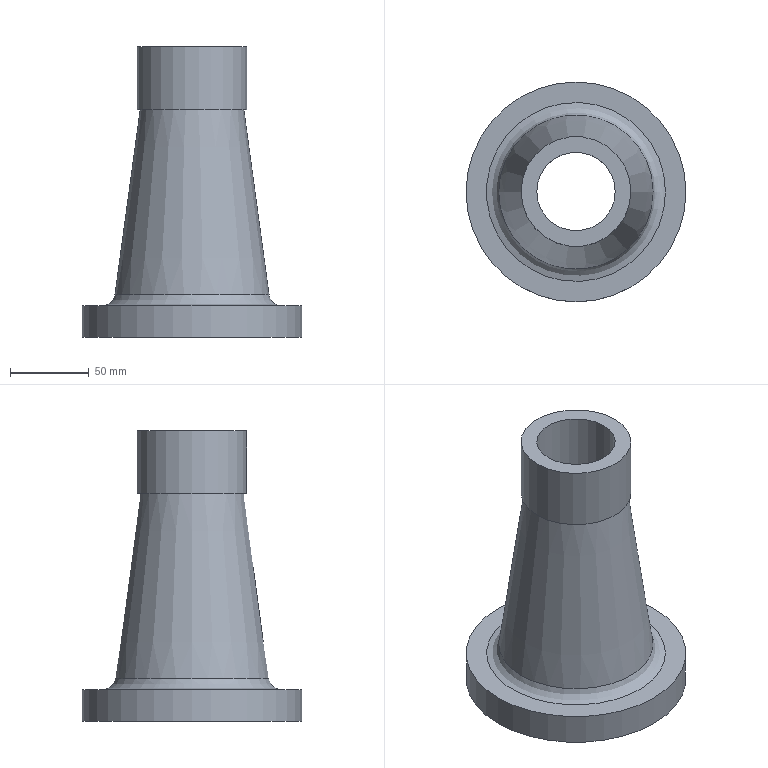Component | NX | BODY | 1 solid | 12 faces | box 140 x 140 x 185 mm | volume 559326 mm3 | plane 5 | cylinder 4 | cone 2 | torus 1 | commonest cylinder face diameters 100 x1 140 x1 70 x1 50 x1
STEP:
#1=CARTESIAN_POINT('',(0.,0.,0.));
#2=DIRECTION('',(0.,0.,1.));
#3=DIRECTION('',(1.,0.,0.));
#4=AXIS2_PLACEMENT_3D('',#1,#2,#3);
#5=CARTESIAN_POINT('',(-42.22,240.,3.));
#6=VERTEX_POINT('',#5);
#7=CARTESIAN_POINT('',(0.,240.,3.));
#8=DIRECTION('',(0.,0.,-1.));
#9=DIRECTION('',(-1.,0.,0.));
#10=AXIS2_PLACEMENT_3D('',#7,#8,#9);
#11=CIRCLE('',#10,42.22);
#12=CARTESIAN_POINT('',(0.,240.,129.617));
#13=DIRECTION('',(0.,0.,-1.));
#14=DIRECTION('',(-1.,0.,0.));
#15=AXIS2_PLACEMENT_3D('',#12,#13,#14);
#16=CONICAL_SURFACE('',#15,25.,0.1352);
#17=CARTESIAN_POINT('',(0.,126.617));
#18=DIRECTION('',(1.,0.));
#19=VECTOR('',#18,1.);
#20=LINE('',#17,#19);
#21=(GEOMETRIC_REPRESENTATION_CONTEXT(2)PARAMETRIC_REPRESENTATION_CONTEXT()REPRESENTATION_CONTEXT('',''));
#22=DEFINITIONAL_REPRESENTATION('',(#20),#21);
#23=PCURVE('',#16,#22);
#24=CARTESIAN_POINT('',(0.,282.22,3.));
#25=DIRECTION('',(0.,0.,-1.));
#26=DIRECTION('',(-1.,0.,0.));
#27=AXIS2_PLACEMENT_3D('',#24,#25,#26);
#28=PLANE('',#27);
#29=CARTESIAN_POINT('',(0.,-42.22));
#30=DIRECTION('',(1.,0.));
#31=AXIS2_PLACEMENT_2D('',#29,#30);
#32=CIRCLE('',#31,42.22);
#33=(GEOMETRIC_REPRESENTATION_CONTEXT(2)PARAMETRIC_REPRESENTATION_CONTEXT()REPRESENTATION_CONTEXT('',''));
#34=DEFINITIONAL_REPRESENTATION('',(#32),#33);
#35=PCURVE('',#28,#34);
#36=SURFACE_CURVE('',#11,(#23,#35),.PCURVE_S1.);
#37=EDGE_CURVE('',#6,#6,#36,.T.);
#38=ORIENTED_EDGE('',*,*,#37,.F.);
#39=CARTESIAN_POINT('',(-25.,240.,129.617));
#40=VERTEX_POINT('',#39);
#41=CARTESIAN_POINT('',(-25.,240.,129.617));
#42=CARTESIAN_POINT('',(-42.22,240.,3.));
#43=B_SPLINE_CURVE_WITH_KNOTS('',1,(#41,#42),.UNSPECIFIED.,.F.,.F.,(2,2),(0.,127.783),.PIECEWISE_BEZIER_KNOTS.);
#44=CARTESIAN_POINT('',(0.,0.));
#45=DIRECTION('',(0.,1.));
#46=VECTOR('',#45,1.);
#47=LINE('',#44,#46);
#48=(GEOMETRIC_REPRESENTATION_CONTEXT(2)PARAMETRIC_REPRESENTATION_CONTEXT()REPRESENTATION_CONTEXT('',''));
#49=DEFINITIONAL_REPRESENTATION('',(#47),#48);
#50=PCURVE('',#16,#49);
#51=CARTESIAN_POINT('',(6.283,0.));
#52=DIRECTION('',(0.,1.));
#53=VECTOR('',#52,1.);
#54=LINE('',#51,#53);
#55=(GEOMETRIC_REPRESENTATION_CONTEXT(2)PARAMETRIC_REPRESENTATION_CONTEXT()REPRESENTATION_CONTEXT('',''));
#56=DEFINITIONAL_REPRESENTATION('',(#54),#55);
#57=PCURVE('',#16,#56);
#58=SEAM_CURVE('',#43,(#50,#57),.PCURVE_S1.);
#59=EDGE_CURVE('',#40,#6,#58,.T.);
#60=ORIENTED_EDGE('',*,*,#59,.F.);
#61=CARTESIAN_POINT('',(0.,240.,129.617));
#62=DIRECTION('',(0.,0.,-1.));
#63=DIRECTION('',(-1.,0.,0.));
#64=AXIS2_PLACEMENT_3D('',#61,#62,#63);
#65=CIRCLE('',#64,25.);
#66=CARTESIAN_POINT('',(0.,0.));
#67=DIRECTION('',(1.,0.));
#68=VECTOR('',#67,1.);
#69=LINE('',#66,#68);
#70=(GEOMETRIC_REPRESENTATION_CONTEXT(2)PARAMETRIC_REPRESENTATION_CONTEXT()REPRESENTATION_CONTEXT('',''));
#71=DEFINITIONAL_REPRESENTATION('',(#69),#70);
#72=PCURVE('',#16,#71);
#73=CARTESIAN_POINT('',(0.,240.,0.));
#74=DIRECTION('',(0.,0.,-1.));
#75=DIRECTION('',(-1.,0.,0.));
#76=AXIS2_PLACEMENT_3D('',#73,#74,#75);
#77=CYLINDRICAL_SURFACE('',#76,25.);
#78=CARTESIAN_POINT('',(0.,-129.617));
#79=DIRECTION('',(1.,0.));
#80=VECTOR('',#79,1.);
#81=LINE('',#78,#80);
#82=(GEOMETRIC_REPRESENTATION_CONTEXT(2)PARAMETRIC_REPRESENTATION_CONTEXT()REPRESENTATION_CONTEXT('',''));
#83=DEFINITIONAL_REPRESENTATION('',(#81),#82);
#84=PCURVE('',#77,#83);
#85=SURFACE_CURVE('',#65,(#72,#84),.PCURVE_S1.);
#86=EDGE_CURVE('',#40,#40,#85,.T.);
#87=ORIENTED_EDGE('',*,*,#86,.T.);
#88=ORIENTED_EDGE('',*,*,#59,.T.);
#89=EDGE_LOOP('',(#38,#60,#87,#88));
#90=FACE_BOUND('',#89,.F.);
#91=ADVANCED_FACE('',(#90),#16,.F.);
#92=CARTESIAN_POINT('',(-50.,240.,3.));
#93=VERTEX_POINT('',#92);
#94=CARTESIAN_POINT('',(0.,240.,3.));
#95=DIRECTION('',(0.,0.,-1.));
#96=DIRECTION('',(-1.,0.,0.));
#97=AXIS2_PLACEMENT_3D('',#94,#95,#96);
#98=CIRCLE('',#97,50.);
#99=CARTESIAN_POINT('',(0.,-42.22));
#100=DIRECTION('',(1.,0.));
#101=AXIS2_PLACEMENT_2D('',#99,#100);
#102=CIRCLE('',#101,50.);
#103=(GEOMETRIC_REPRESENTATION_CONTEXT(2)PARAMETRIC_REPRESENTATION_CONTEXT()REPRESENTATION_CONTEXT('',''));
#104=DEFINITIONAL_REPRESENTATION('',(#102),#103);
#105=PCURVE('',#28,#104);
#106=CARTESIAN_POINT('',(0.,240.,0.));
#107=DIRECTION('',(0.,0.,-1.));
#108=DIRECTION('',(-1.,0.,0.));
#109=AXIS2_PLACEMENT_3D('',#106,#107,#108);
#110=CYLINDRICAL_SURFACE('',#109,50.);
#111=CARTESIAN_POINT('',(0.,-3.));
#112=DIRECTION('',(1.,0.));
#113=VECTOR('',#112,1.);
#114=LINE('',#111,#113);
#115=(GEOMETRIC_REPRESENTATION_CONTEXT(2)PARAMETRIC_REPRESENTATION_CONTEXT()REPRESENTATION_CONTEXT('',''));
#116=DEFINITIONAL_REPRESENTATION('',(#114),#115);
#117=PCURVE('',#110,#116);
#118=SURFACE_CURVE('',#98,(#105,#117),.PCURVE_S1.);
#119=EDGE_CURVE('',#93,#93,#118,.T.);
#120=ORIENTED_EDGE('',*,*,#119,.T.);
#121=EDGE_LOOP('',(#120));
#122=FACE_BOUND('',#121,.T.);
#123=ORIENTED_EDGE('',*,*,#37,.F.);
#124=EDGE_LOOP('',(#123));
#125=FACE_BOUND('',#124,.T.);
#126=ADVANCED_FACE('',(#122,#125),#28,.T.);
#127=CARTESIAN_POINT('',(-50.,240.,0.));
#128=VERTEX_POINT('',#127);
#129=CARTESIAN_POINT('',(0.,240.,0.));
#130=DIRECTION('',(0.,0.,-1.));
#131=DIRECTION('',(-1.,0.,0.));
#132=AXIS2_PLACEMENT_3D('',#129,#130,#131);
#133=CIRCLE('',#132,50.);
#134=CARTESIAN_POINT('',(0.,0.));
#135=DIRECTION('',(1.,0.));
#136=VECTOR('',#135,1.);
#137=LINE('',#134,#136);
#138=(GEOMETRIC_REPRESENTATION_CONTEXT(2)PARAMETRIC_REPRESENTATION_CONTEXT()REPRESENTATION_CONTEXT('',''));
#139=DEFINITIONAL_REPRESENTATION('',(#137),#138);
#140=PCURVE('',#110,#139);
#141=CARTESIAN_POINT('',(0.,290.,0.));
#142=DIRECTION('',(0.,0.,-1.));
#143=DIRECTION('',(-1.,0.,0.));
#144=AXIS2_PLACEMENT_3D('',#141,#142,#143);
#145=PLANE('',#144);
#146=CARTESIAN_POINT('',(0.,-50.));
#147=DIRECTION('',(1.,0.));
#148=AXIS2_PLACEMENT_2D('',#146,#147);
#149=CIRCLE('',#148,50.);
#150=(GEOMETRIC_REPRESENTATION_CONTEXT(2)PARAMETRIC_REPRESENTATION_CONTEXT()REPRESENTATION_CONTEXT('',''));
#151=DEFINITIONAL_REPRESENTATION('',(#149),#150);
#152=PCURVE('',#145,#151);
#153=SURFACE_CURVE('',#133,(#140,#152),.PCURVE_S1.);
#154=EDGE_CURVE('',#128,#128,#153,.T.);
#155=ORIENTED_EDGE('',*,*,#154,.F.);
#156=CARTESIAN_POINT('',(-50.,240.,3.));
#157=CARTESIAN_POINT('',(-50.,240.,0.));
#158=B_SPLINE_CURVE_WITH_KNOTS('',1,(#156,#157),.UNSPECIFIED.,.F.,.F.,(2,2),(-3.,0.),.PIECEWISE_BEZIER_KNOTS.);
#159=CARTESIAN_POINT('',(0.,0.));
#160=DIRECTION('',(0.,1.));
#161=VECTOR('',#160,1.);
#162=LINE('',#159,#161);
#163=(GEOMETRIC_REPRESENTATION_CONTEXT(2)PARAMETRIC_REPRESENTATION_CONTEXT()REPRESENTATION_CONTEXT('',''));
#164=DEFINITIONAL_REPRESENTATION('',(#162),#163);
#165=PCURVE('',#110,#164);
#166=CARTESIAN_POINT('',(6.283,0.));
#167=DIRECTION('',(0.,1.));
#168=VECTOR('',#167,1.);
#169=LINE('',#166,#168);
#170=(GEOMETRIC_REPRESENTATION_CONTEXT(2)PARAMETRIC_REPRESENTATION_CONTEXT()REPRESENTATION_CONTEXT('',''));
#171=DEFINITIONAL_REPRESENTATION('',(#169),#170);
#172=PCURVE('',#110,#171);
#173=SEAM_CURVE('',#158,(#165,#172),.PCURVE_S1.);
#174=EDGE_CURVE('',#93,#128,#173,.T.);
#175=ORIENTED_EDGE('',*,*,#174,.F.);
#176=ORIENTED_EDGE('',*,*,#119,.T.);
#177=ORIENTED_EDGE('',*,*,#174,.T.);
#178=EDGE_LOOP('',(#155,#175,#176,#177));
#179=FACE_BOUND('',#178,.F.);
#180=ADVANCED_FACE('',(#179),#110,.F.);
#181=CARTESIAN_POINT('',(-70.,240.,0.));
#182=VERTEX_POINT('',#181);
#183=CARTESIAN_POINT('',(0.,240.,0.));
#184=DIRECTION('',(0.,0.,-1.));
#185=DIRECTION('',(-1.,0.,0.));
#186=AXIS2_PLACEMENT_3D('',#183,#184,#185);
#187=CIRCLE('',#186,70.);
#188=CARTESIAN_POINT('',(0.,-50.));
#189=DIRECTION('',(1.,0.));
#190=AXIS2_PLACEMENT_2D('',#188,#189);
#191=CIRCLE('',#190,70.);
#192=(GEOMETRIC_REPRESENTATION_CONTEXT(2)PARAMETRIC_REPRESENTATION_CONTEXT()REPRESENTATION_CONTEXT('',''));
#193=DEFINITIONAL_REPRESENTATION('',(#191),#192);
#194=PCURVE('',#145,#193);
#195=CARTESIAN_POINT('',(0.,240.,0.));
#196=DIRECTION('',(0.,0.,-1.));
#197=DIRECTION('',(-1.,0.,0.));
#198=AXIS2_PLACEMENT_3D('',#195,#196,#197);
#199=CYLINDRICAL_SURFACE('',#198,70.);
#200=CARTESIAN_POINT('',(0.,0.));
#201=DIRECTION('',(1.,0.));
#202=VECTOR('',#201,1.);
#203=LINE('',#200,#202);
#204=(GEOMETRIC_REPRESENTATION_CONTEXT(2)PARAMETRIC_REPRESENTATION_CONTEXT()REPRESENTATION_CONTEXT('',''));
#205=DEFINITIONAL_REPRESENTATION('',(#203),#204);
#206=PCURVE('',#199,#205);
#207=SURFACE_CURVE('',#187,(#194,#206),.PCURVE_S1.);
#208=EDGE_CURVE('',#182,#182,#207,.T.);
#209=ORIENTED_EDGE('',*,*,#208,.T.);
#210=EDGE_LOOP('',(#209));
#211=FACE_BOUND('',#210,.T.);
#212=ORIENTED_EDGE('',*,*,#154,.F.);
#213=EDGE_LOOP('',(#212));
#214=FACE_BOUND('',#213,.T.);
#215=ADVANCED_FACE('',(#211,#214),#145,.T.);
#216=CARTESIAN_POINT('',(-70.,240.,20.));
#217=VERTEX_POINT('',#216);
#218=CARTESIAN_POINT('',(0.,240.,20.));
#219=DIRECTION('',(0.,0.,-1.));
#220=DIRECTION('',(-1.,0.,0.));
#221=AXIS2_PLACEMENT_3D('',#218,#219,#220);
#222=CIRCLE('',#221,70.);
#223=CARTESIAN_POINT('',(0.,-20.));
#224=DIRECTION('',(1.,0.));
#225=VECTOR('',#224,1.);
#226=LINE('',#223,#225);
#227=(GEOMETRIC_REPRESENTATION_CONTEXT(2)PARAMETRIC_REPRESENTATION_CONTEXT()REPRESENTATION_CONTEXT('',''));
#228=DEFINITIONAL_REPRESENTATION('',(#226),#227);
#229=PCURVE('',#199,#228);
#230=CARTESIAN_POINT('',(0.,310.,20.));
#231=DIRECTION('',(0.,0.,1.));
#232=DIRECTION('',(1.,0.,0.));
#233=AXIS2_PLACEMENT_3D('',#230,#231,#232);
#234=PLANE('',#233);
#235=CARTESIAN_POINT('',(-70.,-70.));
#236=CARTESIAN_POINT('',(-70.,51.244));
#237=CARTESIAN_POINT('',(35.,-9.378));
#238=CARTESIAN_POINT('',(140.,-70.));
#239=CARTESIAN_POINT('',(35.,-130.622));
#240=CARTESIAN_POINT('',(-70.,-191.244));
#241=CARTESIAN_POINT('',(-70.,-70.));
#242=(BOUNDED_CURVE()B_SPLINE_CURVE(2,(#235,#236,#237,#238,#239,#240,#241),.UNSPECIFIED.,.T.,.F.)B_SPLINE_CURVE_WITH_KNOTS((1,2,2,2,2,1),(-2.094,0.,2.094,4.189,6.283,8.378),.UNSPECIFIED.)CURVE()GEOMETRIC_REPRESENTATION_ITEM()RATIONAL_B_SPLINE_CURVE((1.,0.5,1.,0.5,1.,0.5,1.))REPRESENTATION_ITEM(''));
#243=(GEOMETRIC_REPRESENTATION_CONTEXT(2)PARAMETRIC_REPRESENTATION_CONTEXT()REPRESENTATION_CONTEXT('',''));
#244=DEFINITIONAL_REPRESENTATION('',(#242),#243);
#245=PCURVE('',#234,#244);
#246=SURFACE_CURVE('',#222,(#229,#245),.PCURVE_S1.);
#247=EDGE_CURVE('',#217,#217,#246,.T.);
#248=ORIENTED_EDGE('',*,*,#247,.T.);
#249=CARTESIAN_POINT('',(-70.,240.,20.));
#250=CARTESIAN_POINT('',(-70.,240.,0.));
#251=B_SPLINE_CURVE_WITH_KNOTS('',1,(#249,#250),.UNSPECIFIED.,.F.,.F.,(2,2),(-20.,0.),.PIECEWISE_BEZIER_KNOTS.);
#252=CARTESIAN_POINT('',(6.283,0.));
#253=DIRECTION('',(0.,1.));
#254=VECTOR('',#253,1.);
#255=LINE('',#252,#254);
#256=(GEOMETRIC_REPRESENTATION_CONTEXT(2)PARAMETRIC_REPRESENTATION_CONTEXT()REPRESENTATION_CONTEXT('',''));
#257=DEFINITIONAL_REPRESENTATION('',(#255),#256);
#258=PCURVE('',#199,#257);
#259=CARTESIAN_POINT('',(0.,0.));
#260=DIRECTION('',(0.,1.));
#261=VECTOR('',#260,1.);
#262=LINE('',#259,#261);
#263=(GEOMETRIC_REPRESENTATION_CONTEXT(2)PARAMETRIC_REPRESENTATION_CONTEXT()REPRESENTATION_CONTEXT('',''));
#264=DEFINITIONAL_REPRESENTATION('',(#262),#263);
#265=PCURVE('',#199,#264);
#266=SEAM_CURVE('',#251,(#258,#265),.PCURVE_S1.);
#267=EDGE_CURVE('',#217,#182,#266,.T.);
#268=ORIENTED_EDGE('',*,*,#267,.T.);
#269=ORIENTED_EDGE('',*,*,#208,.F.);
#270=ORIENTED_EDGE('',*,*,#267,.F.);
#271=EDGE_LOOP('',(#248,#268,#269,#270));
#272=FACE_BOUND('',#271,.T.);
#273=ADVANCED_FACE('',(#272),#199,.T.);
#274=CARTESIAN_POINT('',(56.986,240.,20.));
#275=VERTEX_POINT('',#274);
#276=CARTESIAN_POINT('',(0.,240.,20.));
#277=DIRECTION('',(0.,0.,-1.));
#278=DIRECTION('',(1.,0.,0.));
#279=AXIS2_PLACEMENT_3D('',#276,#277,#278);
#280=CIRCLE('',#279,56.986);
#281=CARTESIAN_POINT('',(56.986,-70.));
#282=CARTESIAN_POINT('',(56.986,-168.702));
#283=CARTESIAN_POINT('',(-28.493,-119.351));
#284=CARTESIAN_POINT('',(-113.971,-70.));
#285=CARTESIAN_POINT('',(-28.493,-20.649));
#286=CARTESIAN_POINT('',(56.986,28.702));
#287=CARTESIAN_POINT('',(56.986,-70.));
#288=(BOUNDED_CURVE()B_SPLINE_CURVE(2,(#281,#282,#283,#284,#285,#286,#287),.UNSPECIFIED.,.T.,.F.)B_SPLINE_CURVE_WITH_KNOTS((1,2,2,2,2,1),(-2.094,0.,2.094,4.189,6.283,8.378),.UNSPECIFIED.)CURVE()GEOMETRIC_REPRESENTATION_ITEM()RATIONAL_B_SPLINE_CURVE((1.,0.5,1.,0.5,1.,0.5,1.))REPRESENTATION_ITEM(''));
#289=(GEOMETRIC_REPRESENTATION_CONTEXT(2)PARAMETRIC_REPRESENTATION_CONTEXT()REPRESENTATION_CONTEXT('',''));
#290=DEFINITIONAL_REPRESENTATION('',(#288),#289);
#291=PCURVE('',#234,#290);
#292=CARTESIAN_POINT('',(0.,240.,28.));
#293=DIRECTION('',(0.,0.,1.));
#294=DIRECTION('',(1.,0.,0.));
#295=AXIS2_PLACEMENT_3D('',#292,#293,#294);
#296=TOROIDAL_SURFACE('',#295,56.986,8.);
#297=CARTESIAN_POINT('',(6.283,4.712));
#298=DIRECTION('',(-1.,0.));
#299=VECTOR('',#298,1.);
#300=LINE('',#297,#299);
#301=(GEOMETRIC_REPRESENTATION_CONTEXT(2)PARAMETRIC_REPRESENTATION_CONTEXT()REPRESENTATION_CONTEXT('',''));
#302=DEFINITIONAL_REPRESENTATION('',(#300),#301);
#303=PCURVE('',#296,#302);
#304=SURFACE_CURVE('',#280,(#291,#303),.PCURVE_S1.);
#305=EDGE_CURVE('',#275,#275,#304,.T.);
#306=ORIENTED_EDGE('',*,*,#305,.T.);
#307=EDGE_LOOP('',(#306));
#308=FACE_BOUND('',#307,.T.);
#309=ORIENTED_EDGE('',*,*,#247,.F.);
#310=EDGE_LOOP('',(#309));
#311=FACE_BOUND('',#310,.T.);
#312=ADVANCED_FACE('',(#308,#311),#234,.T.);
#313=CARTESIAN_POINT('',(-49.059,240.,26.922));
#314=VERTEX_POINT('',#313);
#315=CARTESIAN_POINT('',(49.059,240.,26.922));
#316=VERTEX_POINT('',#315);
#317=CARTESIAN_POINT('',(0.,240.,26.922));
#318=DIRECTION('',(0.,0.,1.));
#319=DIRECTION('',(-1.,0.,0.));
#320=AXIS2_PLACEMENT_3D('',#317,#318,#319);
#321=CIRCLE('',#320,49.059);
#322=CARTESIAN_POINT('',(0.,240.,20.));
#323=DIRECTION('',(0.,0.,-1.));
#324=DIRECTION('',(-1.,0.,0.));
#325=AXIS2_PLACEMENT_3D('',#322,#323,#324);
#326=CONICAL_SURFACE('',#325,50.,0.1352);
#327=CARTESIAN_POINT('',(6.283,-6.922));
#328=DIRECTION('',(-1.,0.));
#329=VECTOR('',#328,1.);
#330=LINE('',#327,#329);
#331=(GEOMETRIC_REPRESENTATION_CONTEXT(2)PARAMETRIC_REPRESENTATION_CONTEXT()REPRESENTATION_CONTEXT('',''));
#332=DEFINITIONAL_REPRESENTATION('',(#330),#331);
#333=PCURVE('',#326,#332);
#334=CARTESIAN_POINT('',(3.142,3.277));
#335=DIRECTION('',(1.,0.));
#336=VECTOR('',#335,1.);
#337=LINE('',#334,#336);
#338=(GEOMETRIC_REPRESENTATION_CONTEXT(2)PARAMETRIC_REPRESENTATION_CONTEXT()REPRESENTATION_CONTEXT('',''));
#339=DEFINITIONAL_REPRESENTATION('',(#337),#338);
#340=PCURVE('',#296,#339);
#341=SURFACE_CURVE('',#321,(#333,#340),.PCURVE_S1.);
#342=EDGE_CURVE('',#314,#316,#341,.T.);
#343=ORIENTED_EDGE('',*,*,#342,.T.);
#344=CARTESIAN_POINT('',(0.,240.,26.922));
#345=DIRECTION('',(0.,0.,1.));
#346=DIRECTION('',(-1.,0.,0.));
#347=AXIS2_PLACEMENT_3D('',#344,#345,#346);
#348=CIRCLE('',#347,49.059);
#349=CARTESIAN_POINT('',(6.283,-6.922));
#350=DIRECTION('',(-1.,0.));
#351=VECTOR('',#350,1.);
#352=LINE('',#349,#351);
#353=(GEOMETRIC_REPRESENTATION_CONTEXT(2)PARAMETRIC_REPRESENTATION_CONTEXT()REPRESENTATION_CONTEXT('',''));
#354=DEFINITIONAL_REPRESENTATION('',(#352),#353);
#355=PCURVE('',#326,#354);
#356=CARTESIAN_POINT('',(-3.142,3.277));
#357=DIRECTION('',(1.,0.));
#358=VECTOR('',#357,1.);
#359=LINE('',#356,#358);
#360=(GEOMETRIC_REPRESENTATION_CONTEXT(2)PARAMETRIC_REPRESENTATION_CONTEXT()REPRESENTATION_CONTEXT('',''));
#361=DEFINITIONAL_REPRESENTATION('',(#359),#360);
#362=PCURVE('',#296,#361);
#363=SURFACE_CURVE('',#348,(#355,#362),.PCURVE_S1.);
#364=EDGE_CURVE('',#316,#314,#363,.T.);
#365=ORIENTED_EDGE('',*,*,#364,.T.);
#366=CARTESIAN_POINT('',(-33.,240.,145.));
#367=VERTEX_POINT('',#366);
#368=CARTESIAN_POINT('',(-33.,240.,145.));
#369=CARTESIAN_POINT('',(-49.059,240.,26.922));
#370=B_SPLINE_CURVE_WITH_KNOTS('',1,(#368,#369),.UNSPECIFIED.,.F.,.F.,(2,2),(-126.151,-6.986),.PIECEWISE_BEZIER_KNOTS.);
#371=CARTESIAN_POINT('',(0.,0.));
#372=DIRECTION('',(0.,1.));
#373=VECTOR('',#372,1.);
#374=LINE('',#371,#373);
#375=(GEOMETRIC_REPRESENTATION_CONTEXT(2)PARAMETRIC_REPRESENTATION_CONTEXT()REPRESENTATION_CONTEXT('',''));
#376=DEFINITIONAL_REPRESENTATION('',(#374),#375);
#377=PCURVE('',#326,#376);
#378=CARTESIAN_POINT('',(6.283,0.));
#379=DIRECTION('',(0.,1.));
#380=VECTOR('',#379,1.);
#381=LINE('',#378,#380);
#382=(GEOMETRIC_REPRESENTATION_CONTEXT(2)PARAMETRIC_REPRESENTATION_CONTEXT()REPRESENTATION_CONTEXT('',''));
#383=DEFINITIONAL_REPRESENTATION('',(#381),#382);
#384=PCURVE('',#326,#383);
#385=SEAM_CURVE('',#370,(#377,#384),.PCURVE_S1.);
#386=EDGE_CURVE('',#367,#314,#385,.T.);
#387=ORIENTED_EDGE('',*,*,#386,.F.);
#388=CARTESIAN_POINT('',(0.,240.,145.));
#389=DIRECTION('',(0.,0.,-1.));
#390=DIRECTION('',(-1.,0.,0.));
#391=AXIS2_PLACEMENT_3D('',#388,#389,#390);
#392=CIRCLE('',#391,33.);
#393=CARTESIAN_POINT('',(0.,-125.));
#394=DIRECTION('',(1.,0.));
#395=VECTOR('',#394,1.);
#396=LINE('',#393,#395);
#397=(GEOMETRIC_REPRESENTATION_CONTEXT(2)PARAMETRIC_REPRESENTATION_CONTEXT()REPRESENTATION_CONTEXT('',''));
#398=DEFINITIONAL_REPRESENTATION('',(#396),#397);
#399=PCURVE('',#326,#398);
#400=CARTESIAN_POINT('',(0.,273.,145.));
#401=DIRECTION('',(0.,0.,-1.));
#402=DIRECTION('',(-1.,0.,0.));
#403=AXIS2_PLACEMENT_3D('',#400,#401,#402);
#404=PLANE('',#403);
#405=CARTESIAN_POINT('',(0.,-33.));
#406=DIRECTION('',(1.,0.));
#407=AXIS2_PLACEMENT_2D('',#405,#406);
#408=CIRCLE('',#407,33.);
#409=(GEOMETRIC_REPRESENTATION_CONTEXT(2)PARAMETRIC_REPRESENTATION_CONTEXT()REPRESENTATION_CONTEXT('',''));
#410=DEFINITIONAL_REPRESENTATION('',(#408),#409);
#411=PCURVE('',#404,#410);
#412=SURFACE_CURVE('',#392,(#399,#411),.PCURVE_S1.);
#413=EDGE_CURVE('',#367,#367,#412,.T.);
#414=ORIENTED_EDGE('',*,*,#413,.T.);
#415=ORIENTED_EDGE('',*,*,#386,.T.);
#416=EDGE_LOOP('',(#343,#365,#387,#414,#415));
#417=FACE_BOUND('',#416,.T.);
#418=ADVANCED_FACE('',(#417),#326,.T.);
#419=CARTESIAN_POINT('',(-35.,240.,145.));
#420=VERTEX_POINT('',#419);
#421=CARTESIAN_POINT('',(0.,240.,145.));
#422=DIRECTION('',(0.,0.,-1.));
#423=DIRECTION('',(-1.,0.,0.));
#424=AXIS2_PLACEMENT_3D('',#421,#422,#423);
#425=CIRCLE('',#424,35.);
#426=CARTESIAN_POINT('',(0.,-33.));
#427=DIRECTION('',(1.,0.));
#428=AXIS2_PLACEMENT_2D('',#426,#427);
#429=CIRCLE('',#428,35.);
#430=(GEOMETRIC_REPRESENTATION_CONTEXT(2)PARAMETRIC_REPRESENTATION_CONTEXT()REPRESENTATION_CONTEXT('',''));
#431=DEFINITIONAL_REPRESENTATION('',(#429),#430);
#432=PCURVE('',#404,#431);
#433=CARTESIAN_POINT('',(0.,240.,0.));
#434=DIRECTION('',(0.,0.,-1.));
#435=DIRECTION('',(-1.,0.,0.));
#436=AXIS2_PLACEMENT_3D('',#433,#434,#435);
#437=CYLINDRICAL_SURFACE('',#436,35.);
#438=CARTESIAN_POINT('',(0.,-145.));
#439=DIRECTION('',(1.,0.));
#440=VECTOR('',#439,1.);
#441=LINE('',#438,#440);
#442=(GEOMETRIC_REPRESENTATION_CONTEXT(2)PARAMETRIC_REPRESENTATION_CONTEXT()REPRESENTATION_CONTEXT('',''));
#443=DEFINITIONAL_REPRESENTATION('',(#441),#442);
#444=PCURVE('',#437,#443);
#445=SURFACE_CURVE('',#425,(#432,#444),.PCURVE_S1.);
#446=EDGE_CURVE('',#420,#420,#445,.T.);
#447=ORIENTED_EDGE('',*,*,#446,.T.);
#448=EDGE_LOOP('',(#447));
#449=FACE_BOUND('',#448,.T.);
#450=ORIENTED_EDGE('',*,*,#413,.F.);
#451=EDGE_LOOP('',(#450));
#452=FACE_BOUND('',#451,.T.);
#453=ADVANCED_FACE('',(#449,#452),#404,.T.);
#454=CARTESIAN_POINT('',(-35.,240.,185.));
#455=VERTEX_POINT('',#454);
#456=CARTESIAN_POINT('',(0.,240.,185.));
#457=DIRECTION('',(0.,0.,-1.));
#458=DIRECTION('',(-1.,0.,0.));
#459=AXIS2_PLACEMENT_3D('',#456,#457,#458);
#460=CIRCLE('',#459,35.);
#461=CARTESIAN_POINT('',(0.,-185.));
#462=DIRECTION('',(1.,0.));
#463=VECTOR('',#462,1.);
#464=LINE('',#461,#463);
#465=(GEOMETRIC_REPRESENTATION_CONTEXT(2)PARAMETRIC_REPRESENTATION_CONTEXT()REPRESENTATION_CONTEXT('',''));
#466=DEFINITIONAL_REPRESENTATION('',(#464),#465);
#467=PCURVE('',#437,#466);
#468=CARTESIAN_POINT('',(0.,275.,185.));
#469=DIRECTION('',(0.,0.,1.));
#470=DIRECTION('',(1.,0.,0.));
#471=AXIS2_PLACEMENT_3D('',#468,#469,#470);
#472=PLANE('',#471);
#473=CARTESIAN_POINT('',(-35.,-35.));
#474=CARTESIAN_POINT('',(-35.,25.622));
#475=CARTESIAN_POINT('',(17.5,-4.689));
#476=CARTESIAN_POINT('',(70.,-35.));
#477=CARTESIAN_POINT('',(17.5,-65.311));
#478=CARTESIAN_POINT('',(-35.,-95.622));
#479=CARTESIAN_POINT('',(-35.,-35.));
#480=(BOUNDED_CURVE()B_SPLINE_CURVE(2,(#473,#474,#475,#476,#477,#478,#479),.UNSPECIFIED.,.T.,.F.)B_SPLINE_CURVE_WITH_KNOTS((1,2,2,2,2,1),(-2.094,0.,2.094,4.189,6.283,8.378),.UNSPECIFIED.)CURVE()GEOMETRIC_REPRESENTATION_ITEM()RATIONAL_B_SPLINE_CURVE((1.,0.5,1.,0.5,1.,0.5,1.))REPRESENTATION_ITEM(''));
#481=(GEOMETRIC_REPRESENTATION_CONTEXT(2)PARAMETRIC_REPRESENTATION_CONTEXT()REPRESENTATION_CONTEXT('',''));
#482=DEFINITIONAL_REPRESENTATION('',(#480),#481);
#483=PCURVE('',#472,#482);
#484=SURFACE_CURVE('',#460,(#467,#483),.PCURVE_S1.);
#485=EDGE_CURVE('',#455,#455,#484,.T.);
#486=ORIENTED_EDGE('',*,*,#485,.T.);
#487=CARTESIAN_POINT('',(-35.,240.,185.));
#488=CARTESIAN_POINT('',(-35.,240.,145.));
#489=B_SPLINE_CURVE_WITH_KNOTS('',1,(#487,#488),.UNSPECIFIED.,.F.,.F.,(2,2),(-185.,-145.),.PIECEWISE_BEZIER_KNOTS.);
#490=CARTESIAN_POINT('',(6.283,0.));
#491=DIRECTION('',(0.,1.));
#492=VECTOR('',#491,1.);
#493=LINE('',#490,#492);
#494=(GEOMETRIC_REPRESENTATION_CONTEXT(2)PARAMETRIC_REPRESENTATION_CONTEXT()REPRESENTATION_CONTEXT('',''));
#495=DEFINITIONAL_REPRESENTATION('',(#493),#494);
#496=PCURVE('',#437,#495);
#497=CARTESIAN_POINT('',(0.,0.));
#498=DIRECTION('',(0.,1.));
#499=VECTOR('',#498,1.);
#500=LINE('',#497,#499);
#501=(GEOMETRIC_REPRESENTATION_CONTEXT(2)PARAMETRIC_REPRESENTATION_CONTEXT()REPRESENTATION_CONTEXT('',''));
#502=DEFINITIONAL_REPRESENTATION('',(#500),#501);
#503=PCURVE('',#437,#502);
#504=SEAM_CURVE('',#489,(#496,#503),.PCURVE_S1.);
#505=EDGE_CURVE('',#455,#420,#504,.T.);
#506=ORIENTED_EDGE('',*,*,#505,.T.);
#507=ORIENTED_EDGE('',*,*,#446,.F.);
#508=ORIENTED_EDGE('',*,*,#505,.F.);
#509=EDGE_LOOP('',(#486,#506,#507,#508));
#510=FACE_BOUND('',#509,.T.);
#511=ADVANCED_FACE('',(#510),#437,.T.);
#512=CARTESIAN_POINT('',(-25.,240.,185.));
#513=VERTEX_POINT('',#512);
#514=CARTESIAN_POINT('',(0.,240.,185.));
#515=DIRECTION('',(0.,0.,-1.));
#516=DIRECTION('',(-1.,0.,0.));
#517=AXIS2_PLACEMENT_3D('',#514,#515,#516);
#518=CIRCLE('',#517,25.);
#519=CARTESIAN_POINT('',(-25.,-35.));
#520=CARTESIAN_POINT('',(-25.,8.301));
#521=CARTESIAN_POINT('',(12.5,-13.349));
#522=CARTESIAN_POINT('',(50.,-35.));
#523=CARTESIAN_POINT('',(12.5,-56.651));
#524=CARTESIAN_POINT('',(-25.,-78.301));
#525=CARTESIAN_POINT('',(-25.,-35.));
#526=(BOUNDED_CURVE()B_SPLINE_CURVE(2,(#519,#520,#521,#522,#523,#524,#525),.UNSPECIFIED.,.T.,.F.)B_SPLINE_CURVE_WITH_KNOTS((1,2,2,2,2,1),(-2.094,0.,2.094,4.189,6.283,8.378),.UNSPECIFIED.)CURVE()GEOMETRIC_REPRESENTATION_ITEM()RATIONAL_B_SPLINE_CURVE((1.,0.5,1.,0.5,1.,0.5,1.))REPRESENTATION_ITEM(''));
#527=(GEOMETRIC_REPRESENTATION_CONTEXT(2)PARAMETRIC_REPRESENTATION_CONTEXT()REPRESENTATION_CONTEXT('',''));
#528=DEFINITIONAL_REPRESENTATION('',(#526),#527);
#529=PCURVE('',#472,#528);
#530=CARTESIAN_POINT('',(0.,-185.));
#531=DIRECTION('',(1.,0.));
#532=VECTOR('',#531,1.);
#533=LINE('',#530,#532);
#534=(GEOMETRIC_REPRESENTATION_CONTEXT(2)PARAMETRIC_REPRESENTATION_CONTEXT()REPRESENTATION_CONTEXT('',''));
#535=DEFINITIONAL_REPRESENTATION('',(#533),#534);
#536=PCURVE('',#77,#535);
#537=SURFACE_CURVE('',#518,(#529,#536),.PCURVE_S1.);
#538=EDGE_CURVE('',#513,#513,#537,.T.);
#539=ORIENTED_EDGE('',*,*,#538,.T.);
#540=EDGE_LOOP('',(#539));
#541=FACE_BOUND('',#540,.T.);
#542=ORIENTED_EDGE('',*,*,#485,.F.);
#543=EDGE_LOOP('',(#542));
#544=FACE_BOUND('',#543,.T.);
#545=ADVANCED_FACE('',(#541,#544),#472,.T.);
#546=ORIENTED_EDGE('',*,*,#86,.F.);
#547=CARTESIAN_POINT('',(-25.,240.,185.));
#548=CARTESIAN_POINT('',(-25.,240.,129.617));
#549=B_SPLINE_CURVE_WITH_KNOTS('',1,(#547,#548),.UNSPECIFIED.,.F.,.F.,(2,2),(-185.,-129.617),.PIECEWISE_BEZIER_KNOTS.);
#550=CARTESIAN_POINT('',(0.,0.));
#551=DIRECTION('',(0.,1.));
#552=VECTOR('',#551,1.);
#553=LINE('',#550,#552);
#554=(GEOMETRIC_REPRESENTATION_CONTEXT(2)PARAMETRIC_REPRESENTATION_CONTEXT()REPRESENTATION_CONTEXT('',''));
#555=DEFINITIONAL_REPRESENTATION('',(#553),#554);
#556=PCURVE('',#77,#555);
#557=CARTESIAN_POINT('',(6.283,0.));
#558=DIRECTION('',(0.,1.));
#559=VECTOR('',#558,1.);
#560=LINE('',#557,#559);
#561=(GEOMETRIC_REPRESENTATION_CONTEXT(2)PARAMETRIC_REPRESENTATION_CONTEXT()REPRESENTATION_CONTEXT('',''));
#562=DEFINITIONAL_REPRESENTATION('',(#560),#561);
#563=PCURVE('',#77,#562);
#564=SEAM_CURVE('',#549,(#556,#563),.PCURVE_S1.);
#565=EDGE_CURVE('',#513,#40,#564,.T.);
#566=ORIENTED_EDGE('',*,*,#565,.F.);
#567=ORIENTED_EDGE('',*,*,#538,.T.);
#568=ORIENTED_EDGE('',*,*,#565,.T.);
#569=EDGE_LOOP('',(#546,#566,#567,#568));
#570=FACE_BOUND('',#569,.F.);
#571=ADVANCED_FACE('',(#570),#77,.F.);
#572=ORIENTED_EDGE('',*,*,#342,.T.);
#573=CARTESIAN_POINT('',(49.059,240.,26.922));
#574=CARTESIAN_POINT('',(49.321,240.,24.992));
#575=CARTESIAN_POINT('',(50.138,240.,23.18));
#576=CARTESIAN_POINT('',(51.446,240.,21.656));
#577=CARTESIAN_POINT('',(53.132,240.,20.565));
#578=CARTESIAN_POINT('',(55.038,240.,20.));
#579=CARTESIAN_POINT('',(56.986,240.,20.));
#580=(BOUNDED_CURVE()B_SPLINE_CURVE(6,(#573,#574,#575,#576,#577,#578,#579),.UNSPECIFIED.,.F.,.F.)B_SPLINE_CURVE_WITH_KNOTS((7,7),(3.277,4.712),.PIECEWISE_BEZIER_KNOTS.)CURVE()GEOMETRIC_REPRESENTATION_ITEM()RATIONAL_B_SPLINE_CURVE((1.026,1.008,0.9983,0.9949,0.9983,1.008,1.026))REPRESENTATION_ITEM(''));
#581=CARTESIAN_POINT('',(6.283,0.));
#582=DIRECTION('',(0.,1.));
#583=VECTOR('',#582,1.);
#584=LINE('',#581,#583);
#585=(GEOMETRIC_REPRESENTATION_CONTEXT(2)PARAMETRIC_REPRESENTATION_CONTEXT()REPRESENTATION_CONTEXT('',''));
#586=DEFINITIONAL_REPRESENTATION('',(#584),#585);
#587=PCURVE('',#296,#586);
#588=CARTESIAN_POINT('',(0.,0.));
#589=DIRECTION('',(0.,1.));
#590=VECTOR('',#589,1.);
#591=LINE('',#588,#590);
#592=(GEOMETRIC_REPRESENTATION_CONTEXT(2)PARAMETRIC_REPRESENTATION_CONTEXT()REPRESENTATION_CONTEXT('',''));
#593=DEFINITIONAL_REPRESENTATION('',(#591),#592);
#594=PCURVE('',#296,#593);
#595=SEAM_CURVE('',#580,(#587,#594),.PCURVE_S1.);
#596=EDGE_CURVE('',#316,#275,#595,.T.);
#597=ORIENTED_EDGE('',*,*,#596,.T.);
#598=ORIENTED_EDGE('',*,*,#305,.T.);
#599=ORIENTED_EDGE('',*,*,#596,.F.);
#600=ORIENTED_EDGE('',*,*,#364,.T.);
#601=EDGE_LOOP('',(#572,#597,#598,#599,#600));
#602=FACE_BOUND('',#601,.F.);
#603=ADVANCED_FACE('',(#602),#296,.F.);
#604=CLOSED_SHELL('',(#91,#126,#180,#215,#273,#312,#418,#453,#511,#545,#571,#603));
#605=MANIFOLD_SOLID_BREP('',#604);
#606=(LENGTH_UNIT()NAMED_UNIT(*)SI_UNIT(.MILLI.,.METRE.));
#607=UNCERTAINTY_MEASURE_WITH_UNIT(LENGTH_MEASURE(0.00001),#606,'','');
#608=(NAMED_UNIT(*)PLANE_ANGLE_UNIT()SI_UNIT($,.RADIAN.));
#609=(NAMED_UNIT(*)SI_UNIT($,.STERADIAN.)SOLID_ANGLE_UNIT());
#610=(GEOMETRIC_REPRESENTATION_CONTEXT(3)GLOBAL_UNCERTAINTY_ASSIGNED_CONTEXT((#607))GLOBAL_UNIT_ASSIGNED_CONTEXT((#606,#608,#609))REPRESENTATION_CONTEXT('',''));
#611=ADVANCED_BREP_SHAPE_REPRESENTATION('',(#4,#605),#610);